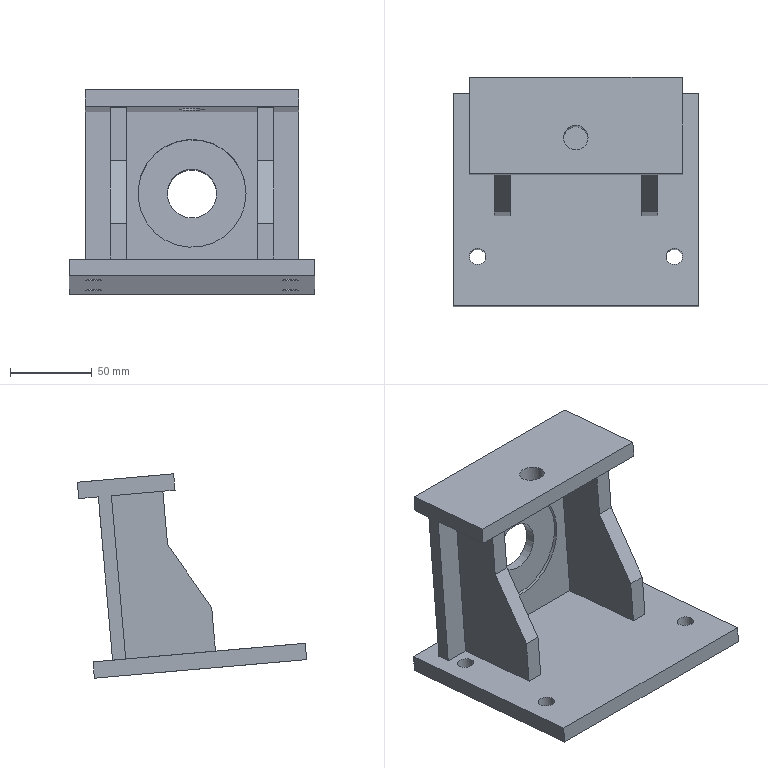Component | NX | FRAME | 1 solid | 36 faces | volume 444835 mm3 | plane 29 | cylinder 7 | commonest cylinder face diameters 10 x4 66 x1 30 x1 15 x1